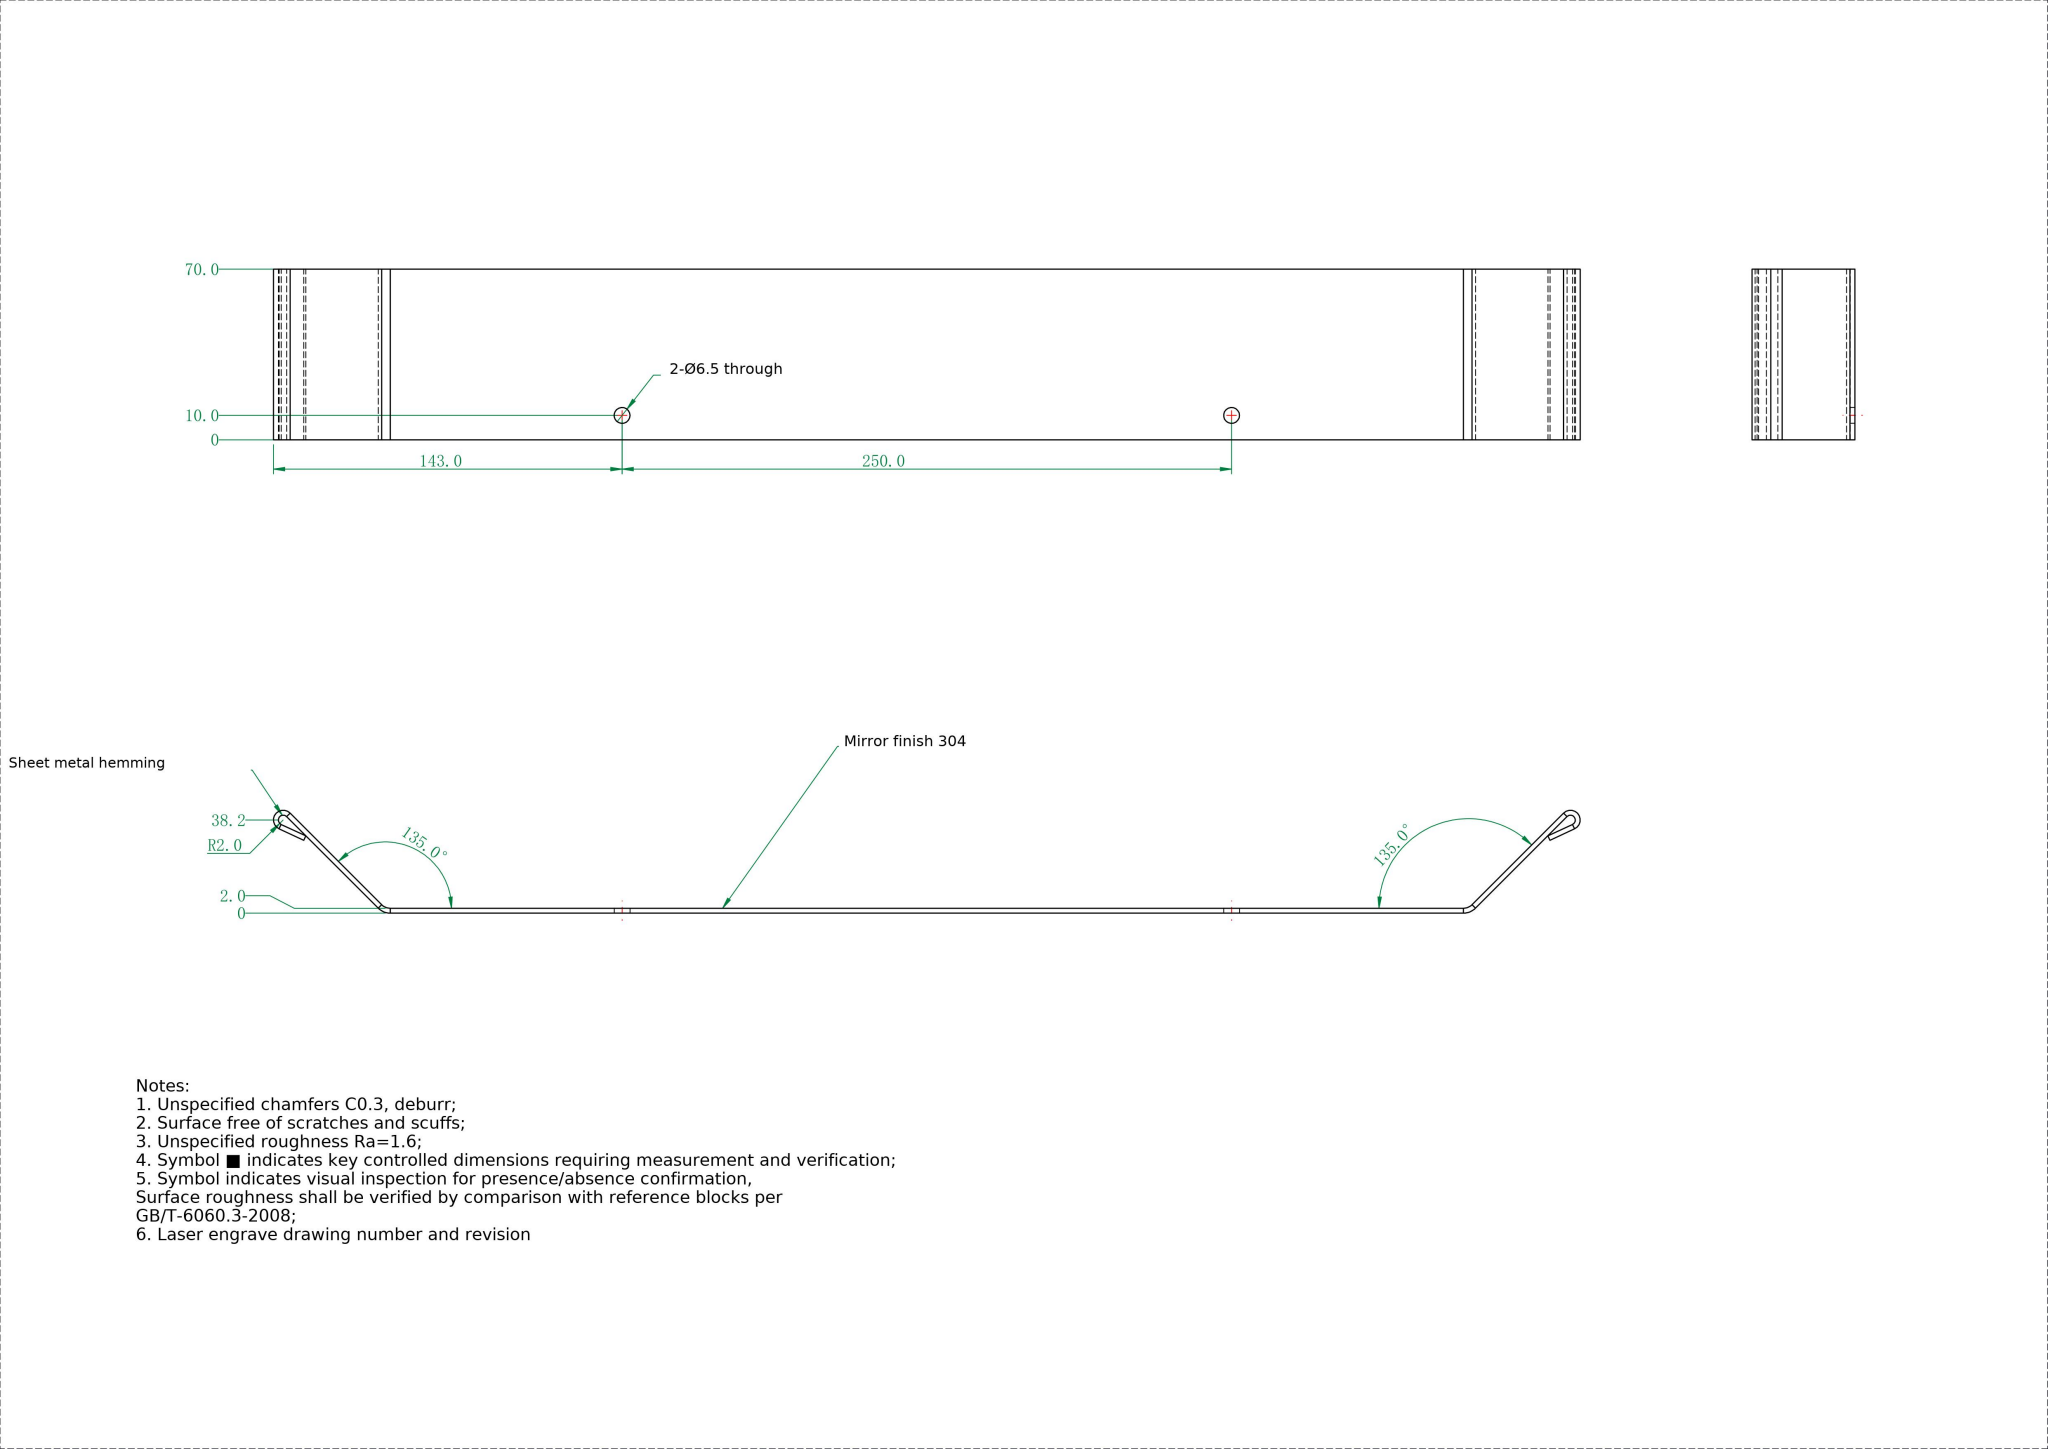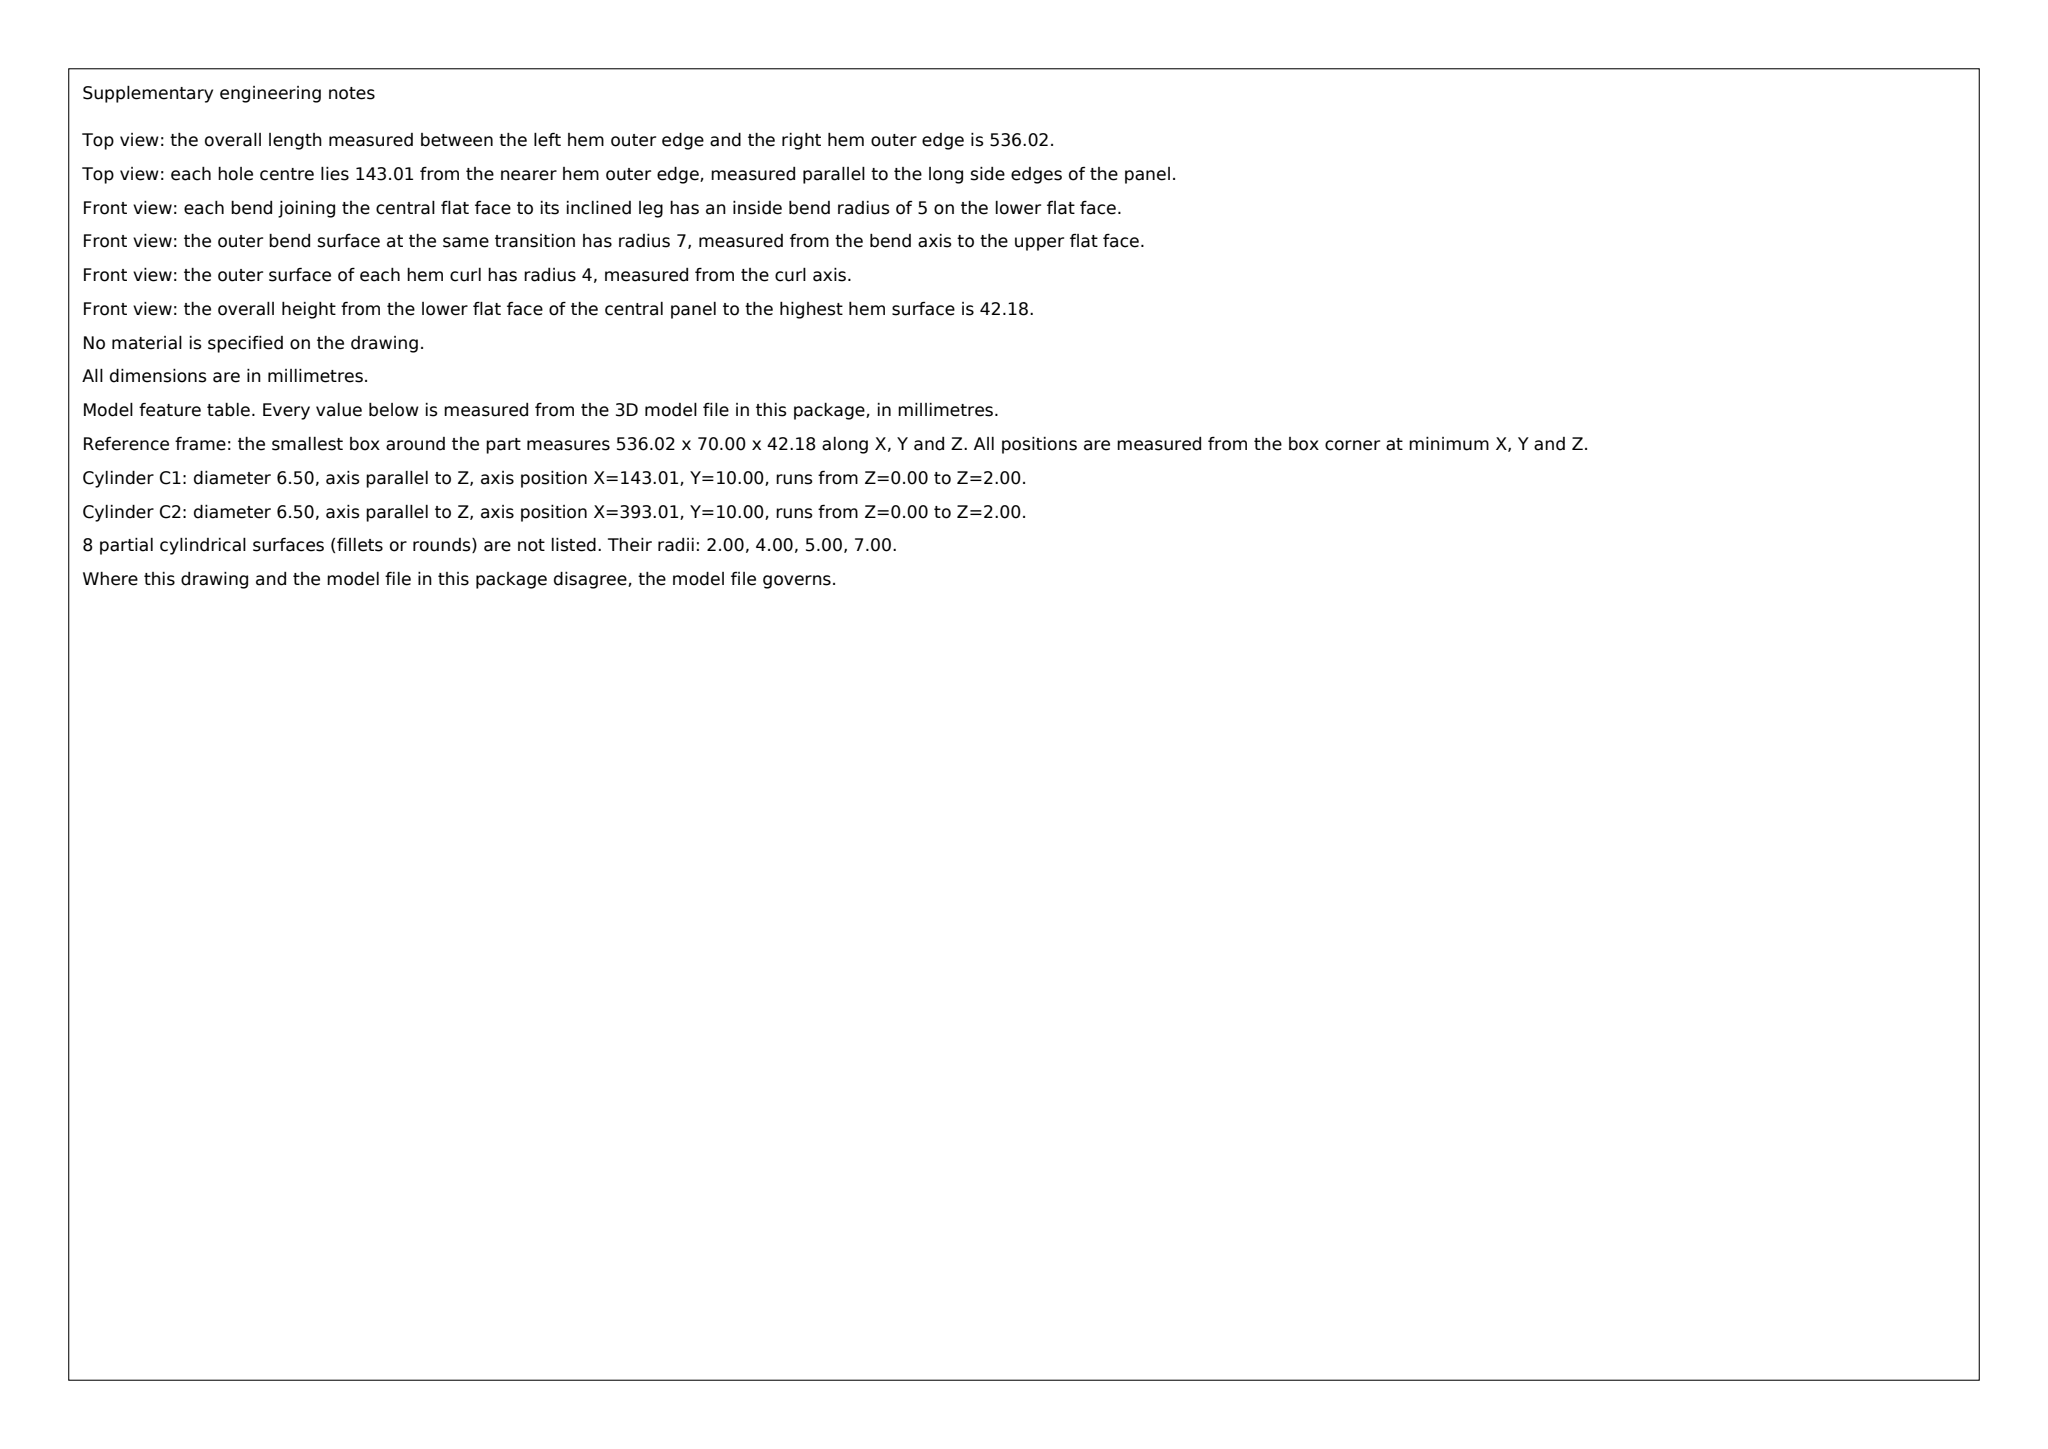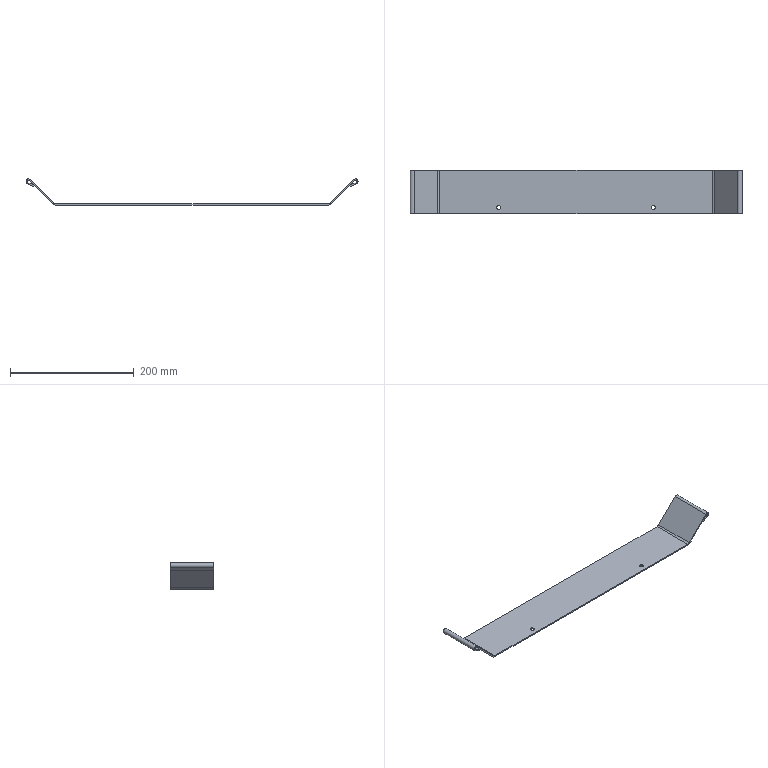Part | SolidWorks | mm | material 304 | 1 solid | 42 faces | box 536.02 x 70 x 42.18 mm | volume 83735 mm3 | plane 30 | cylinder 12 | commonest cylinder face diameters 6.5 x4 14 x2 10 x2 8 x2 4 x2
Drawing notes:
BEND TANGENTS 47.9 & 488.1 FROM LH END; BTM FLAT 440.2 BTWN | from the solid: z=0 plane x[47.9,488.1]; R5/R7 bend arcs at x=47.9 and 488.1; bbox X=536.024
FLANGE 53.0 LG, BEND TANGENT TO HEM CURL CTR, TYP 2 PL | from the solid: 45 deg inclined faces 37.5 x 37.5 in XZ => 53.03 slant; ends at hem ctr (4.0,38.2)
R5.0 BEND & R2.0 HEM TYP BOTH ENDS; PART SYM ABOUT CL | from the solid: concave Ø10 arcs @x=47.9/488.1, convex Ø14; concave Ø4 / convex Ø8 hems @x=4.0/532.0
TEARDROP HEM: 200° CURL R2.0 INR, Ø8.0 OD, TYP 2 PL | from the solid: concave dia 4.0 and convex dia 8.0 arcs, arc_deg 200, axis y at z=38.2
HEM CURL CTR 4.0 FROM PART END, 38.2 ABOVE BTM FLAT, TYP 2 PL | from the solid: hem arc axis_pos [4.0,-,38.2] and [532.0,-,38.2]; bbox X 0-536.024
KEY DIM 11.1 = HEM TAIL FLAT, CURL TANGENT TO SHEET EDGE | from the solid: inclined planes 10.1 x 4.7 at 25° to X => 11.14 flat length, 2.0 apart
HEM TAIL AT 25° TO BTM FLAT; END FACE 2.0 THK, TYP 2 PL | from the solid: inclined_planes angle_to_xyz [65,90,25] size 10.1x4.7; end face 0.8x1.8 = 2.0 thk